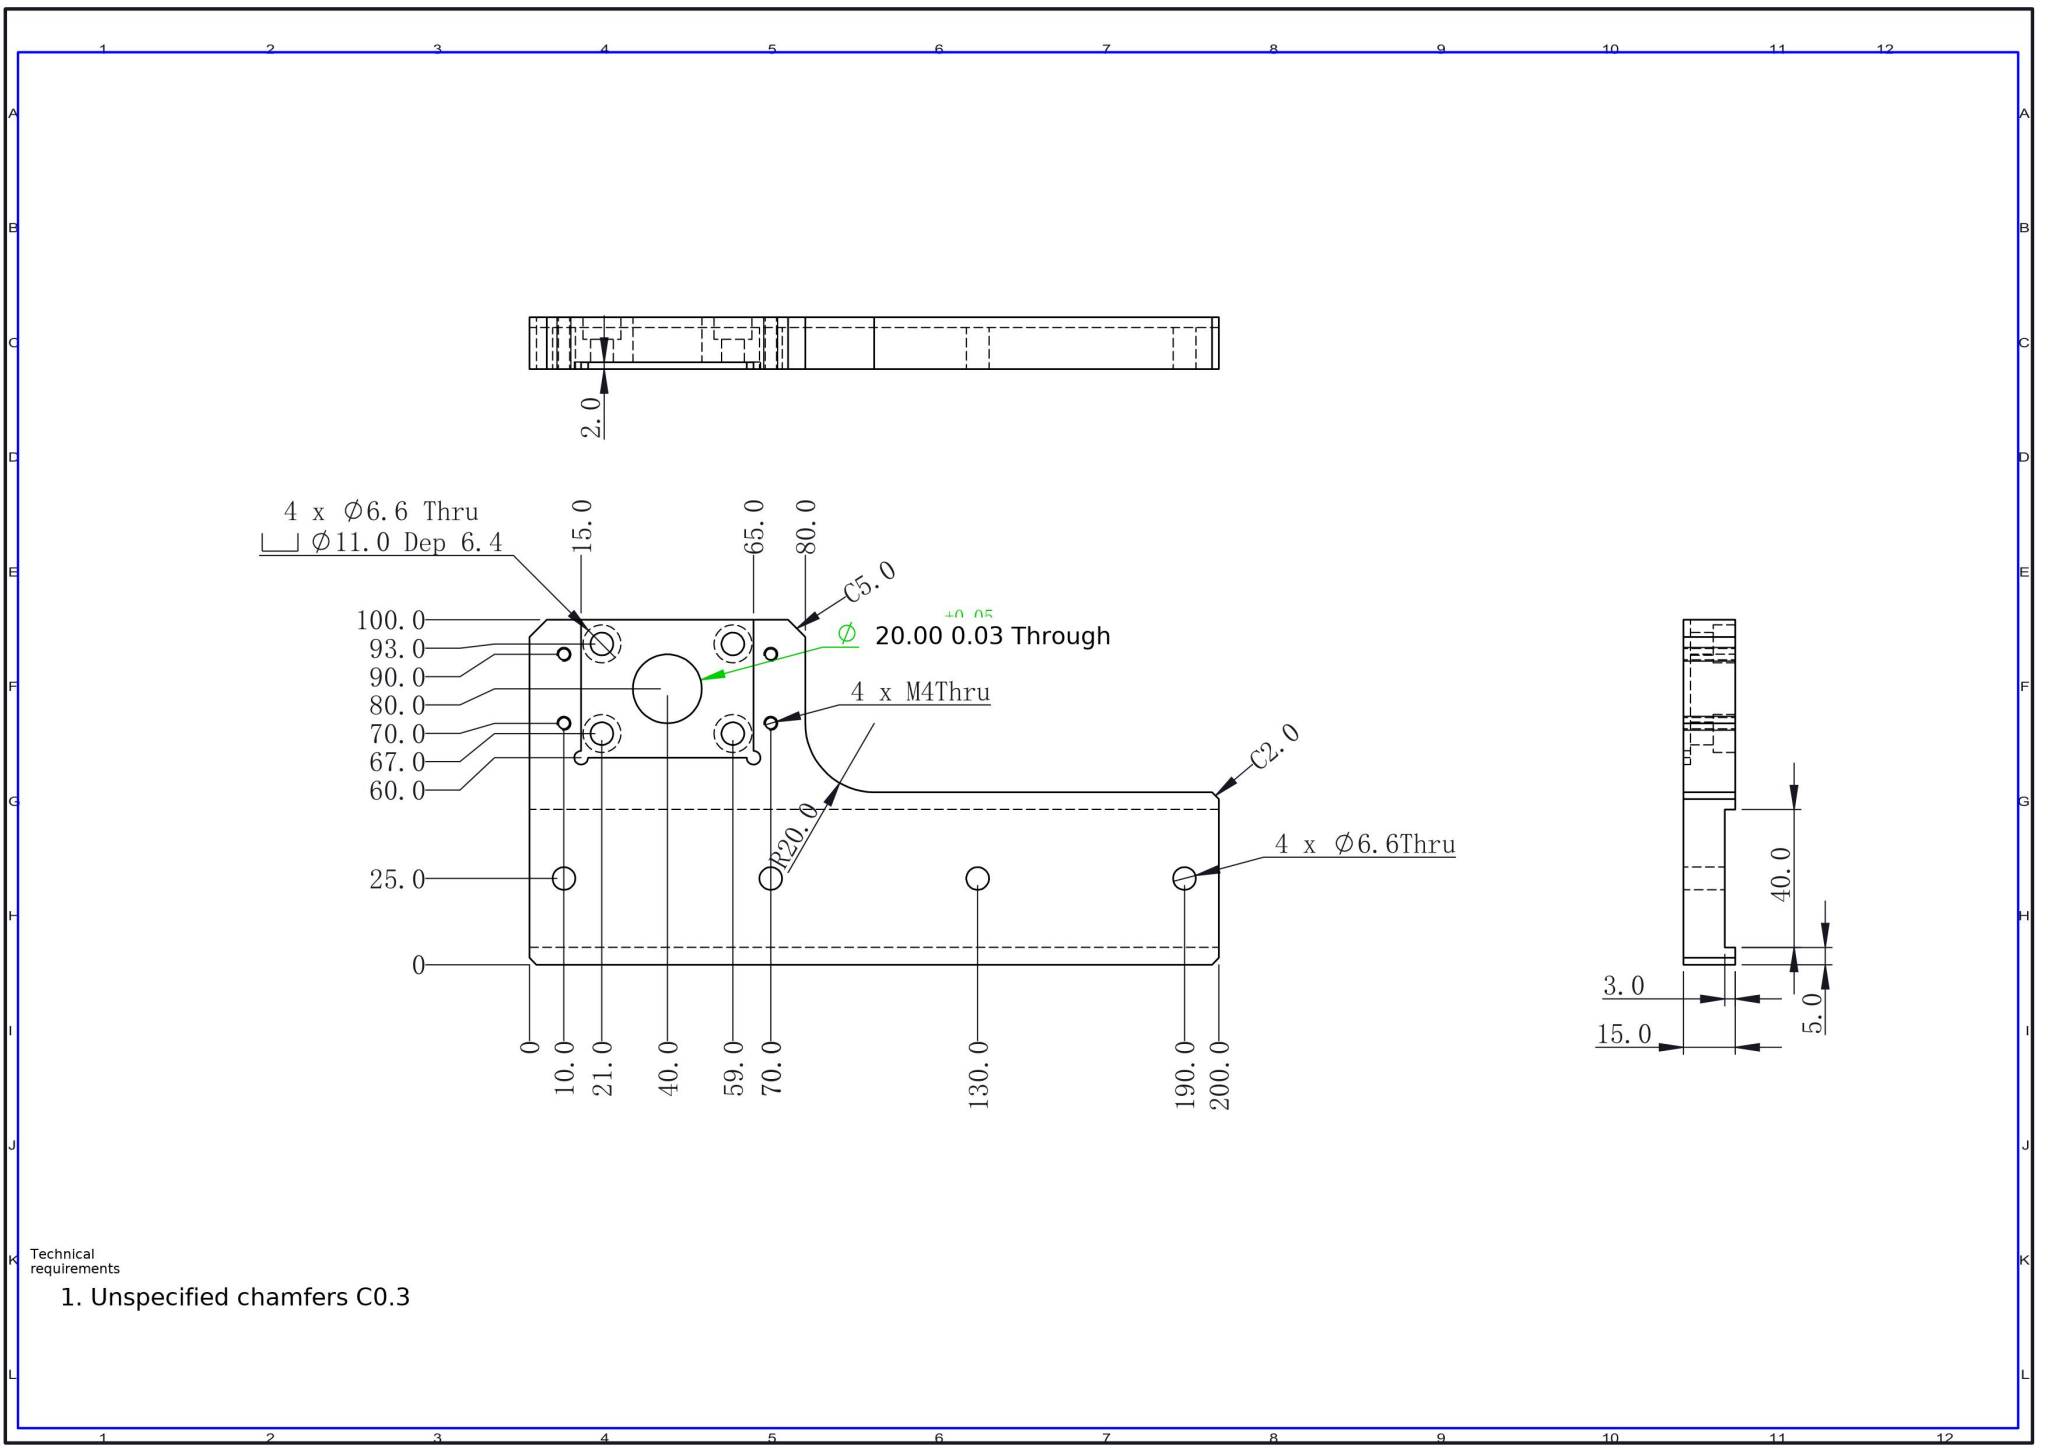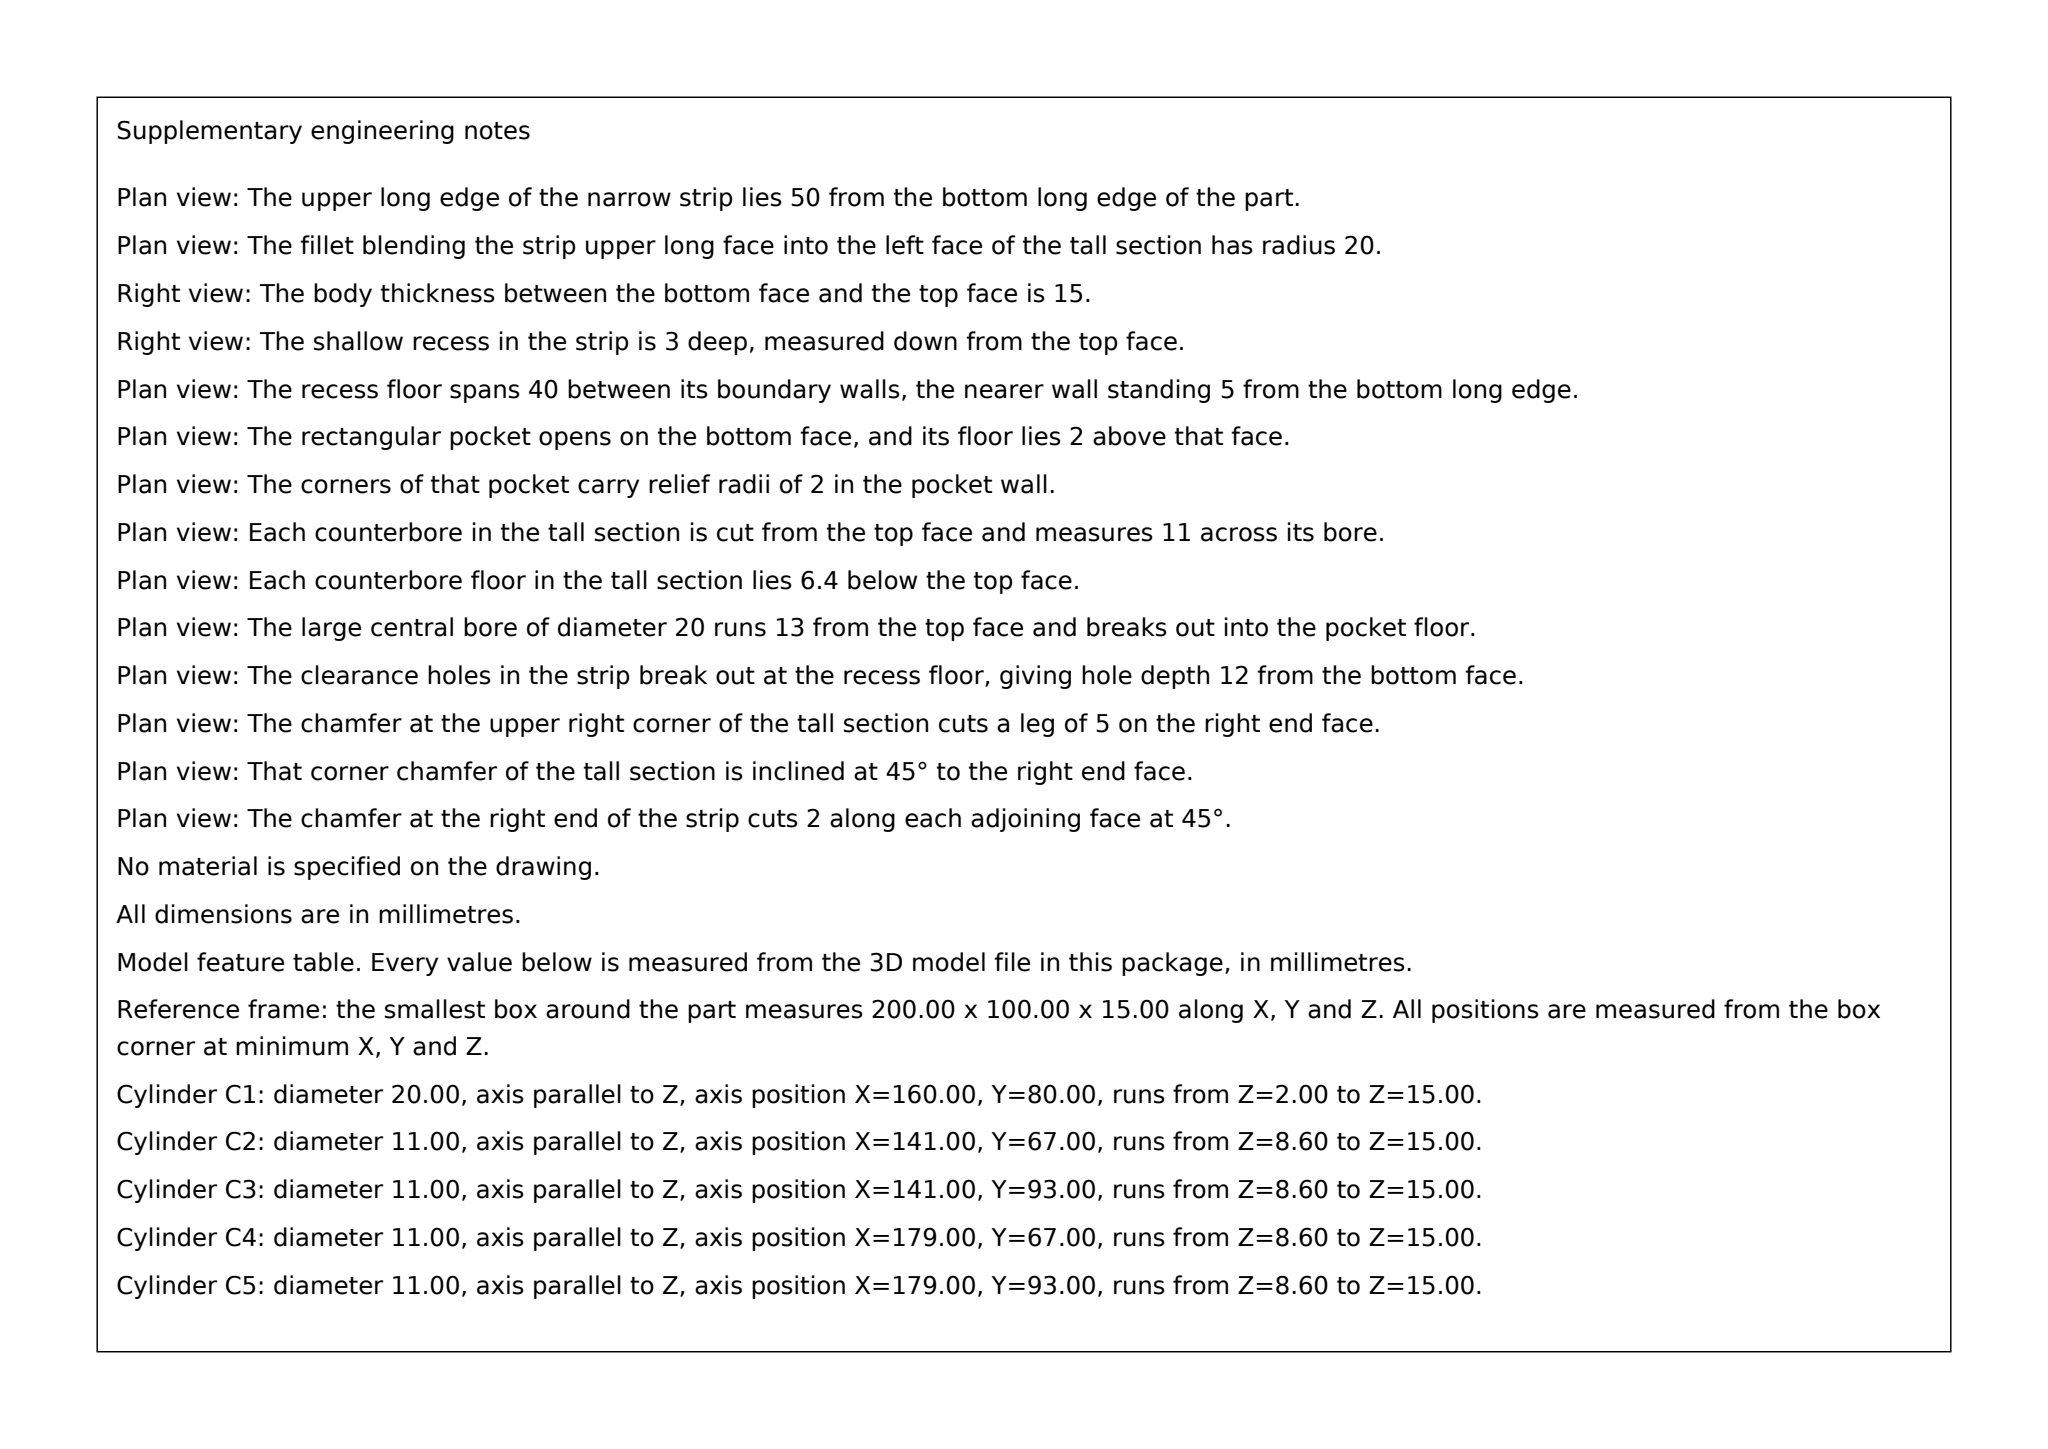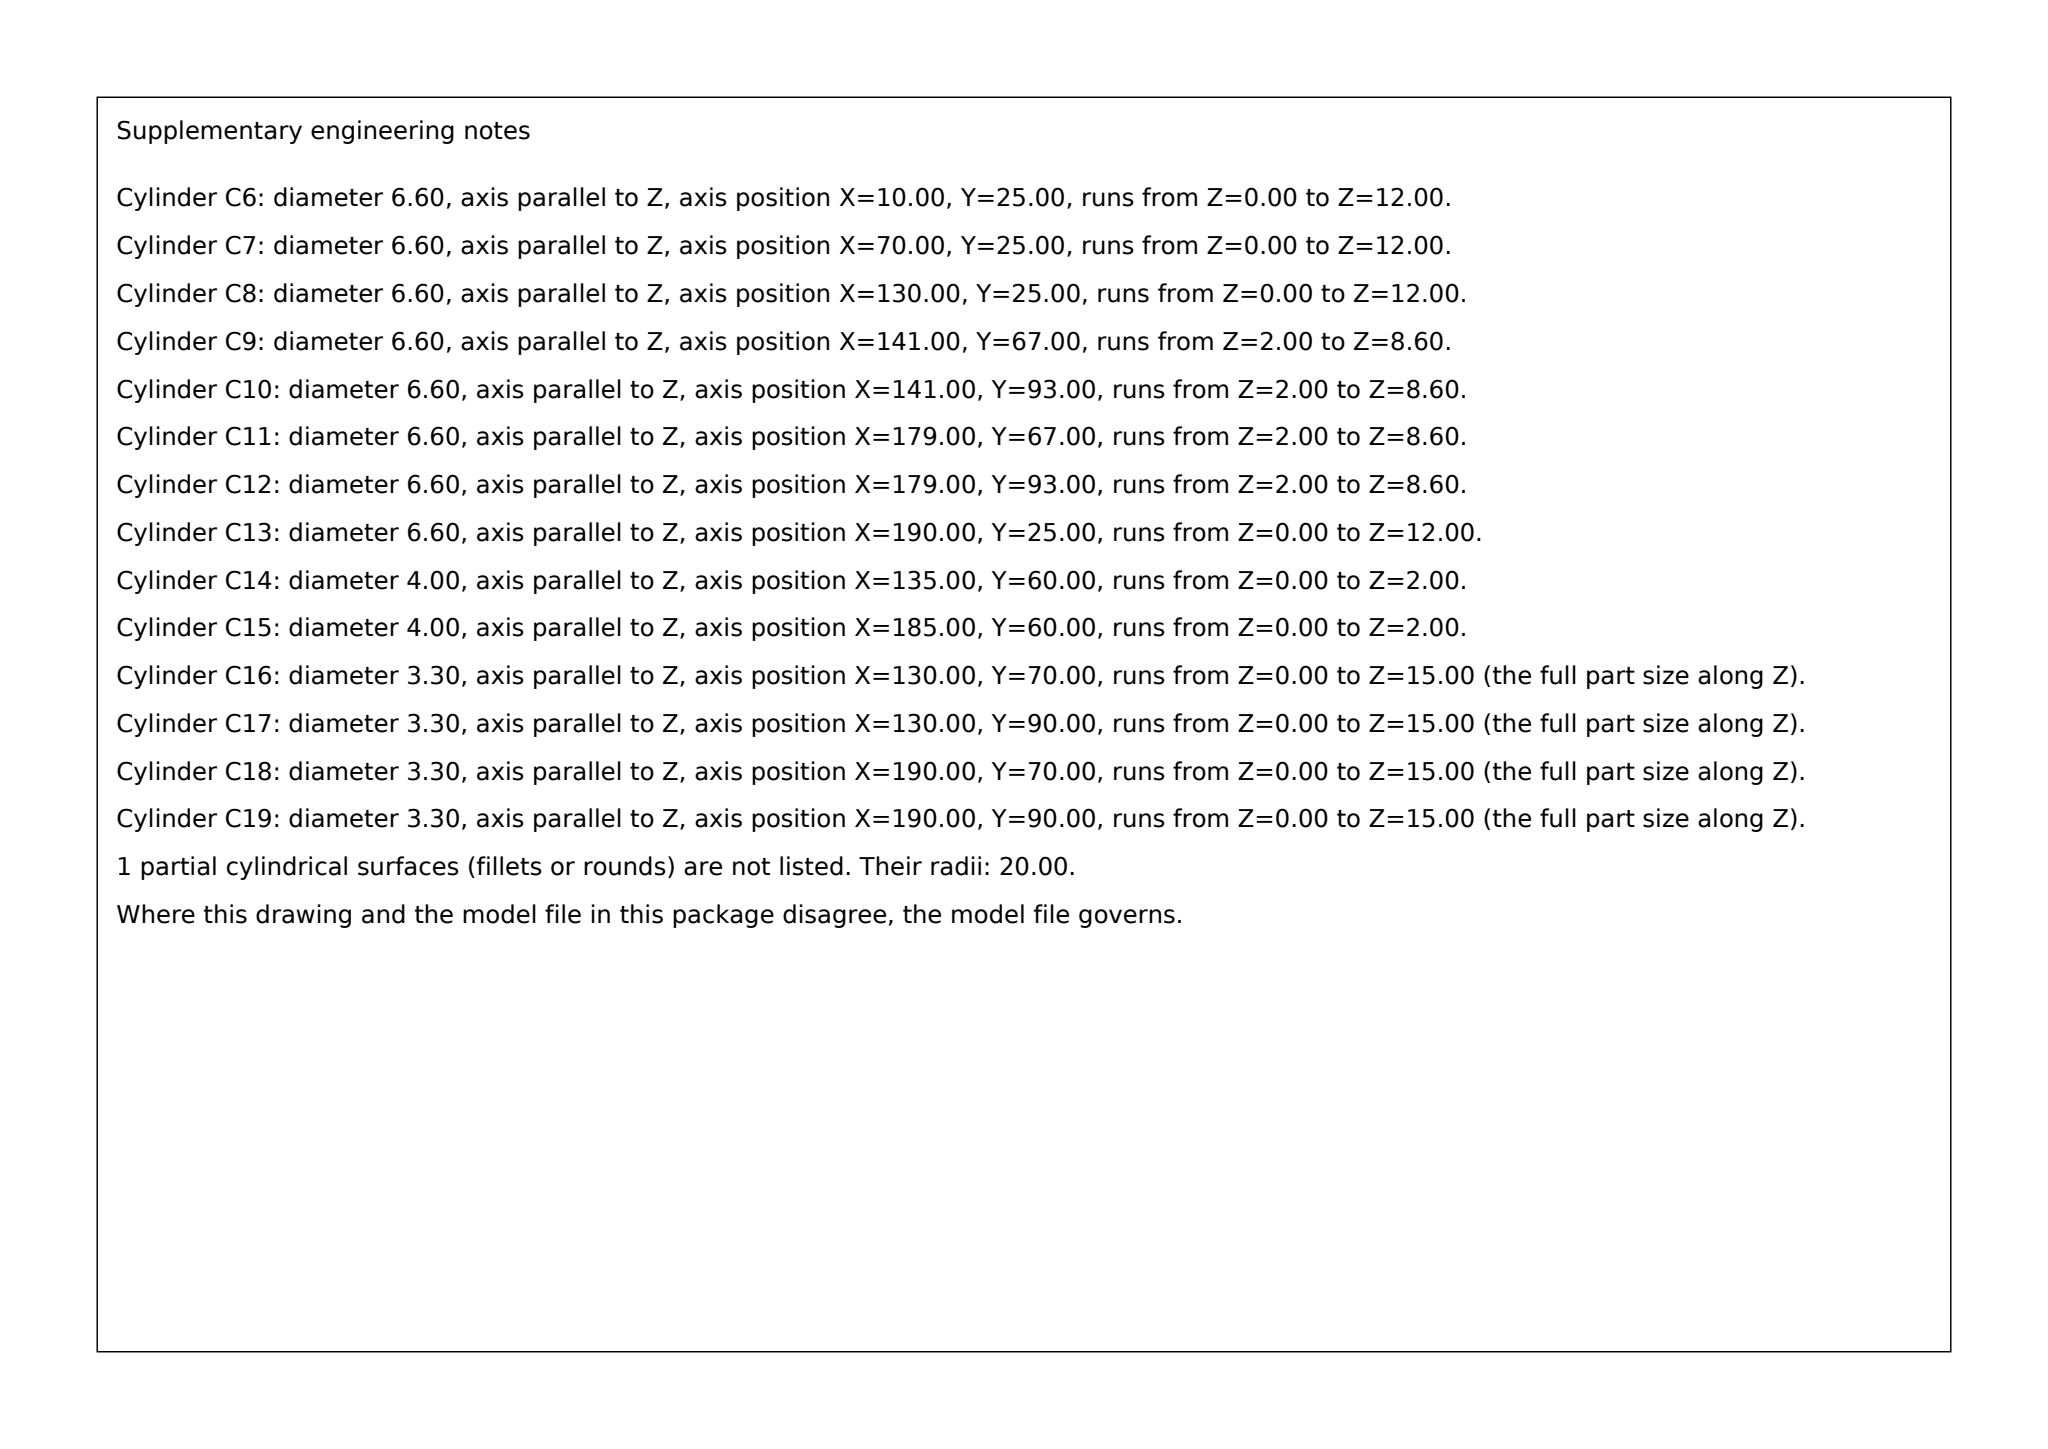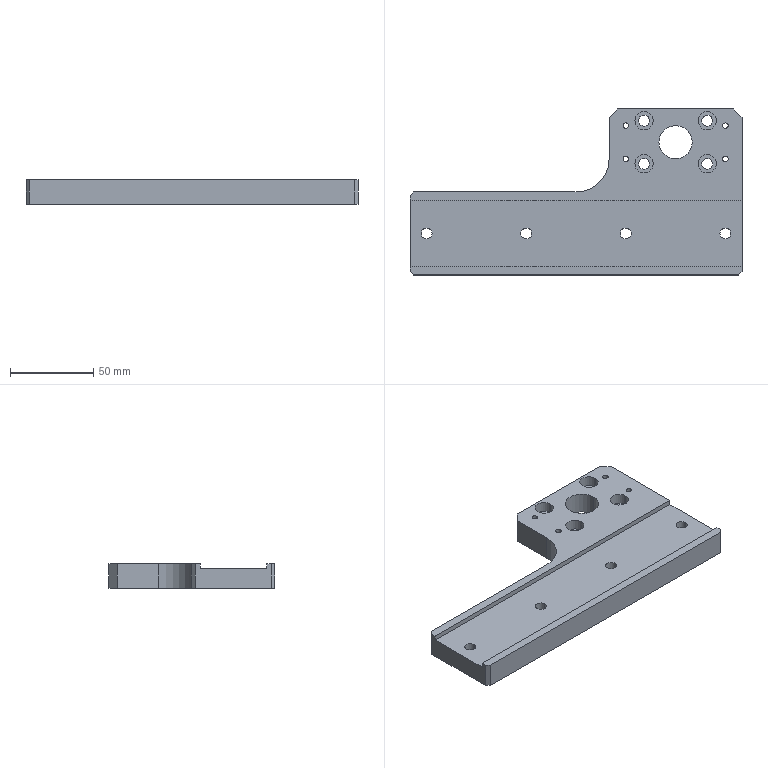Part | SolidWorks | mm | 1 solid | 63 faces | box 200 x 100 x 15 mm | volume 173209 mm3 | cylinder 38 | plane 25 | commonest cylinder face diameters 6.6 x16 3.3 x8 11 x8 4 x3 20 x2 40 x1
Drawing notes:
POCKET 50 WIDE (X15.0-65.0) X 40 (Y60.0-100.0) DP 2.0 | from the solid: z plane 2.0 floor; x planes 135 & 185 = 15.0 & 65.0 from datum (bbox 200); y 60.0 to 100.0 edge; R2 corners from Ø4.0 z-cyls L=2.0 at (135,60) & (185,60); Ø20 thru len 13.0 = 15.0-2.0 confirms depth
build123d program:
from build123d import *

# Parameters (mm, degrees)
BOSS_EXTRUDE1_DEPTH                             = 15
SKETCH2_W                                       = 200
SKETCH2_H                                       = 40
CUT_EXTRUDE1_DEPTH                              = 3
CUT_EXTRUDE2_DEPTH                              = 225.109
CUT_EXTRUDE2_DEPTH_BACK                         = 225.109
SKETCH3_R                                       = 10
M6_HEX_SOCKET_HEAD_CAP_SCREW_CBORE1_D           = 6.6
M6_HEX_SOCKET_HEAD_CAP_SCREW_CBORE1_CBORE_D     = 11
M6_HEX_SOCKET_HEAD_CAP_SCREW_CBORE1_CBORE_DEPTH = 6.4
M4_TAPPED_HOLE1_D                               = 3.3
M6_CLEARANCE_HOLE1_D                            = 6.6
FILLET1_R                                       = 20
CHAMFER1_SIZE                                   = 5
CHAMFER2_SIZE                                   = 2
SKETCH10_W                                      = 50
SKETCH10_H                                      = 40
CUT_EXTRUDE3_DEPTH                              = 2
SKETCH11_R                                      = 2
CUT_EXTRUDE4_DEPTH                              = 2


with BuildPart() as part:
    # Sketch1 → Boss-Extrude1 (new body)
    with BuildSketch(Plane.XY):
        Polygon((0, 0), (200, 0), (200, 100), (120, 100), (120, 50), (0, 50), align=None)
    extrude(amount=BOSS_EXTRUDE1_DEPTH)

    # Sketch2 → Cut-Extrude1 (cut)
    with BuildSketch(Plane(origin=(0, 0, 15), x_dir=(-1, 0, 0), z_dir=(0, 0, -1))):
        with Locations((-100, 25)):
            Rectangle(SKETCH2_W, SKETCH2_H)
    extrude(amount=CUT_EXTRUDE1_DEPTH, mode=Mode.SUBTRACT)

    # Sketch3 → Cut-Extrude2 (cut, two sides: drawn at the far end of the back side and taken through both)
    with BuildSketch(Plane.XY.offset(15).offset(-CUT_EXTRUDE2_DEPTH_BACK)):
        with Locations((160, 80)):
            Circle(SKETCH3_R)
    extrude(amount=CUT_EXTRUDE2_DEPTH + CUT_EXTRUDE2_DEPTH_BACK, mode=Mode.SUBTRACT)

    # M6 Hex Socket Head Cap Screw CBORE1 (through all)
    with Locations(Plane.XY.offset(15)):
        with Locations((141, 93), (179, 93), (179, 67), (141, 67)):
            CounterBoreHole(M6_HEX_SOCKET_HEAD_CAP_SCREW_CBORE1_D / 2, M6_HEX_SOCKET_HEAD_CAP_SCREW_CBORE1_CBORE_D / 2, M6_HEX_SOCKET_HEAD_CAP_SCREW_CBORE1_CBORE_DEPTH)

    # M4 Tapped Hole1 (through all)
    with Locations(Plane.XY.offset(15)):
        with Locations((130, 90), (130, 70), (190, 70), (190, 90)):
            Hole(M4_TAPPED_HOLE1_D / 2)

    # M6 Clearance Hole1 (through all)
    with Locations(Plane.XY.offset(12)):
        with Locations((10, 25), (70, 25), (130, 25), (190, 25)):
            Hole(M6_CLEARANCE_HOLE1_D / 2)

    # Fillet1
    fillet1_edges = [part.edges().sort_by_distance(p)[0] for p in [
        (120, 50, 7.5),
    ]]
    fillet(fillet1_edges, radius=FILLET1_R)

    # Chamfer1
    chamfer1_edges = [part.edges().sort_by_distance(p)[0] for p in [
        (120, 100, 7.5),
        (200, 100, 7.5),
    ]]
    chamfer(chamfer1_edges, length=CHAMFER1_SIZE)

    # Chamfer2
    chamfer2_edges = [part.edges().sort_by_distance(p)[0] for p in [
        (0, 50, 7.5),
        (200, 0, 7.5),
        (0, 0, 7.5),
    ]]
    chamfer(chamfer2_edges, length=CHAMFER2_SIZE)

    # Sketch10 → Cut-Extrude3 (cut)
    with BuildSketch(Plane(origin=(0, 0, 0), x_dir=(-1, 0, 0), z_dir=(0, 0, -1))):
        with Locations((-160, 80)):
            Rectangle(SKETCH10_W, SKETCH10_H)
    extrude(amount=-CUT_EXTRUDE3_DEPTH, mode=Mode.SUBTRACT)

    # Sketch11 → Cut-Extrude4 (cut)
    with BuildSketch(Plane(origin=(0, 0, 0), x_dir=(-1, 0, 0), z_dir=(0, 0, -1))):
        with Locations((-185, 60)):
            Circle(SKETCH11_R)
        with Locations((-135, 60)):
            Circle(SKETCH11_R)
    extrude(amount=-CUT_EXTRUDE4_DEPTH, mode=Mode.SUBTRACT)


solid = part.part